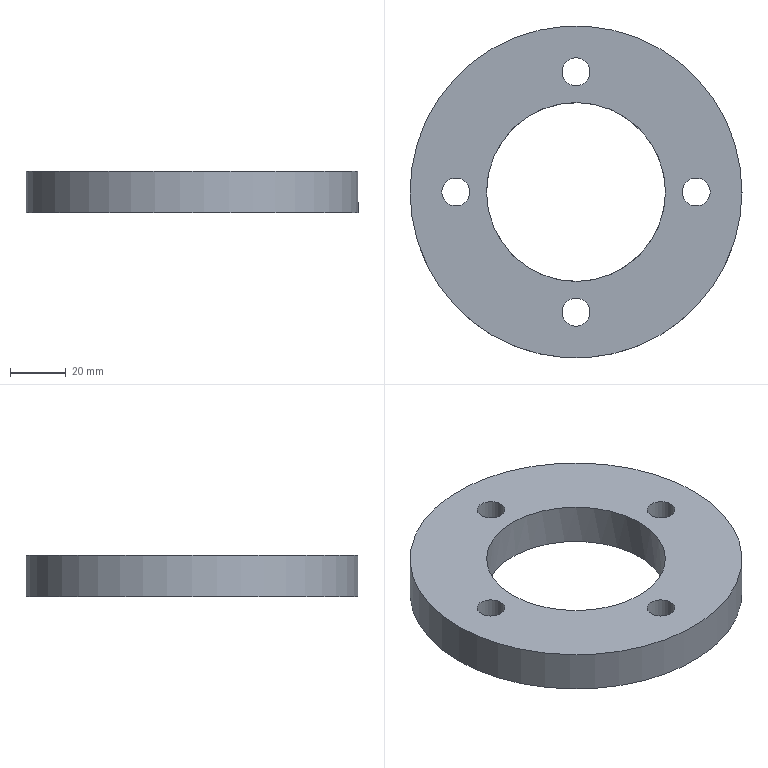Component | NX | ZYC50 | 1 solid | 16 faces | volume 111199 mm3 | cylinder 10 | plane 6 | commonest cylinder face diameters 10 x4 15 x4 118.75 x1 64 x1